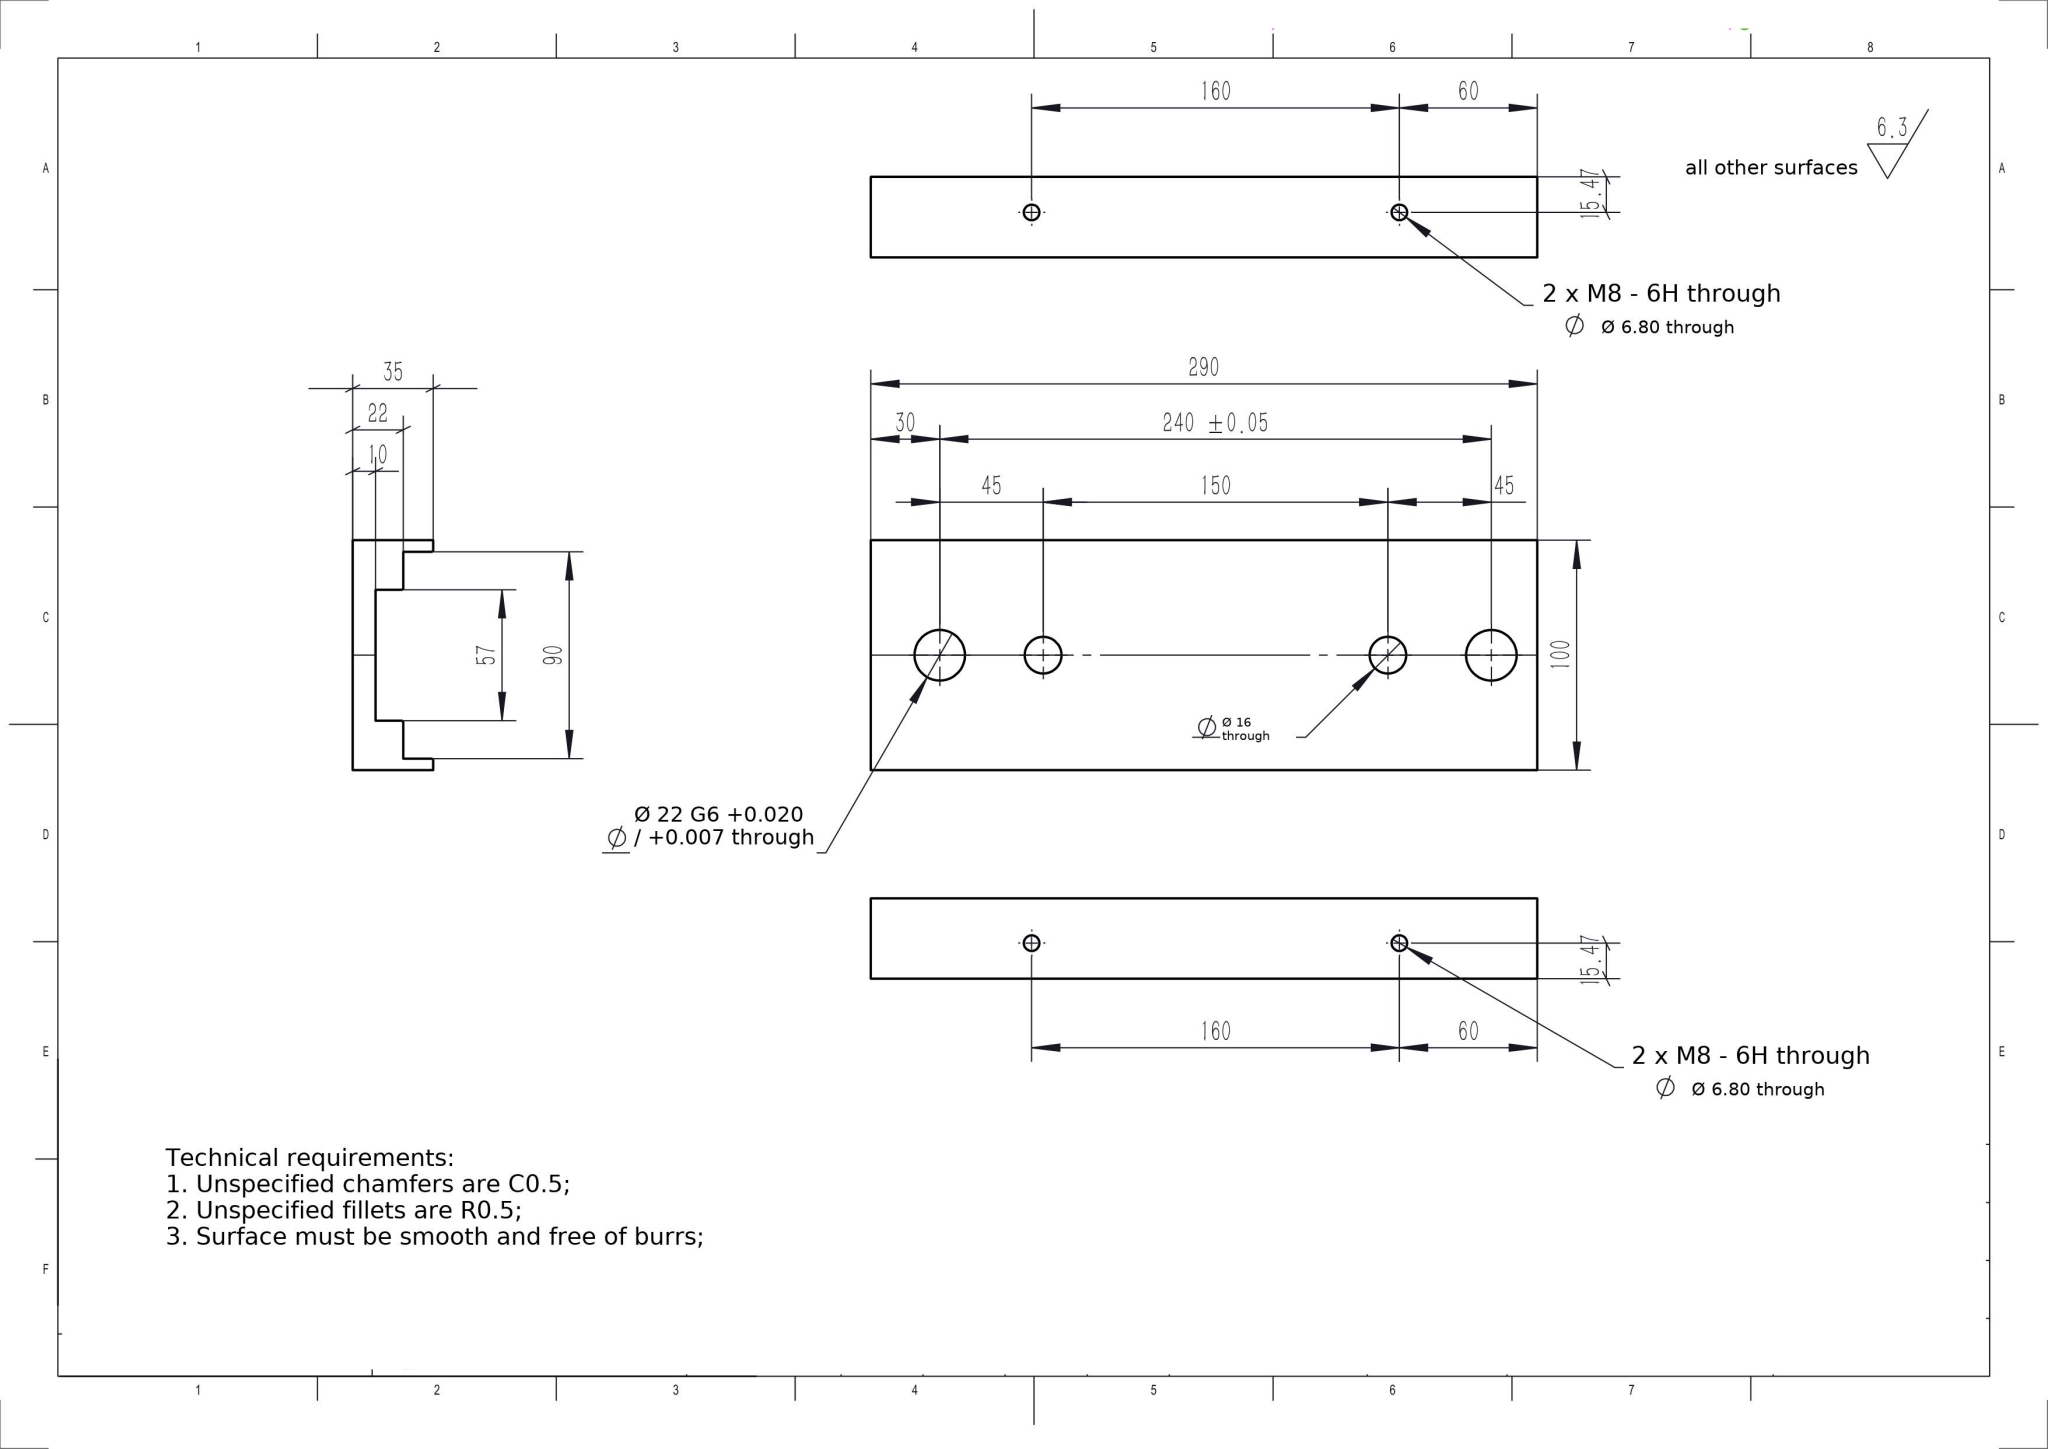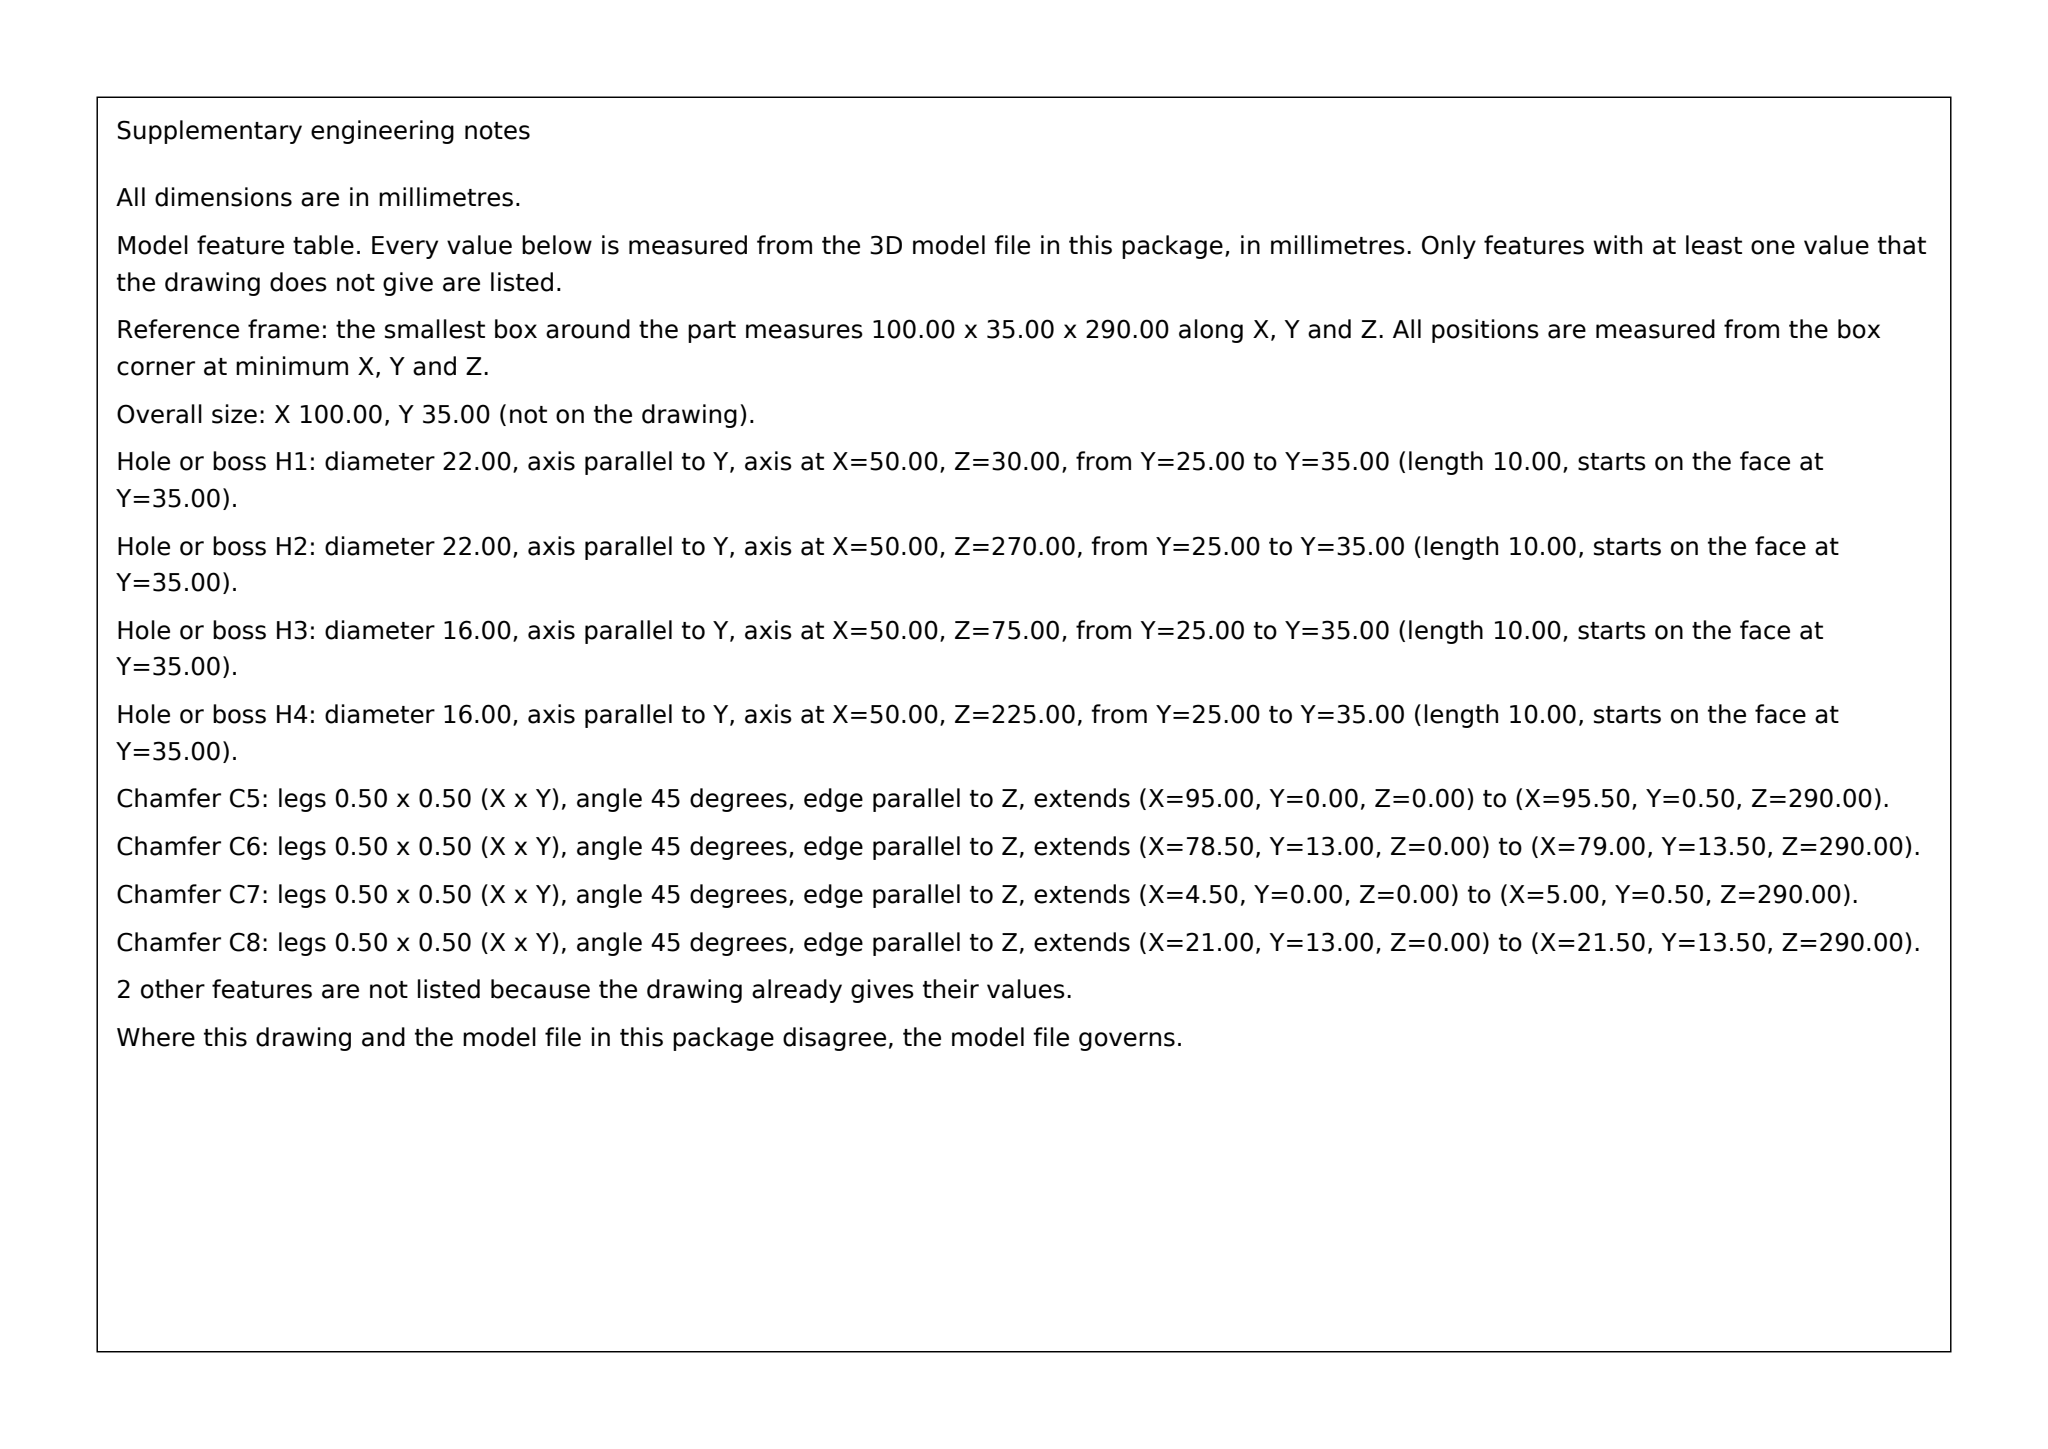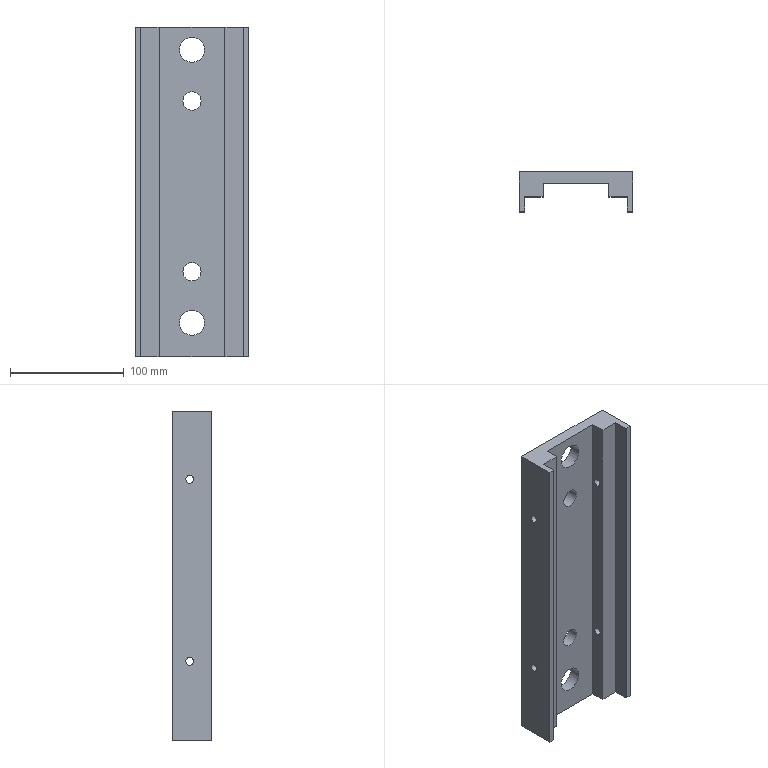Part | SolidWorks | mm | 1 solid | 34 faces | box 100 x 35 x 290 mm | volume 462448 mm3 | plane 18 | cylinder 16 | commonest cylinder face diameters 6.8 x8 22 x4 16 x4
build123d program:
from build123d import *

# Parameters (mm, degrees)
BOSS_EXTRUDE2_DEPTH = 300
SKETCH2_R           = 11
SKETCH2_R_2         = 8
CUT_EXTRUDE1_DEPTH  = 10
M8_TAPPED_HOLE1_D   = 6.8
CHAMFER1_SIZE       = 0.5
SKETCH6_W           = 100
SKETCH6_H           = 10
CUT_EXTRUDE2_DEPTH  = 319.159


with BuildPart() as part:
    # Sketch1 → Boss-Extrude2 (new body)
    with BuildSketch(Plane.XY):
        Polygon((0, 0), (0, 35), (100, 35), (100, 0), (95, 0), (95, 13), (78.5, 13), (78.5, 25), (21.5, 25), (21.5, 13), (5, 13), (5, 0), align=None)
    extrude(amount=BOSS_EXTRUDE2_DEPTH)

    # Sketch2 → Cut-Extrude1 (cut)
    with BuildSketch(Plane(origin=(0, 35, 0), x_dir=(1, 0, 0), z_dir=(0, 1, 0))):
        with Locations(Location((50, -30, 0), (0, 0, 180))):
            Circle(SKETCH2_R)
        with Locations((50, -270)):
            Circle(SKETCH2_R)
        with Locations(Location((50, -75, 0), (0, 0, 180))):
            Circle(SKETCH2_R_2)
        with Locations((50, -225)):
            Circle(SKETCH2_R_2)
    extrude(amount=-CUT_EXTRUDE1_DEPTH, mode=Mode.SUBTRACT)

    # M8 Tapped Hole1 (through all)
    with Locations(Plane(origin=(100, 0, 0), x_dir=(0, 0, -1), z_dir=(1, 0, 0))):
        with Locations((-230, 19.528), (-70, 19.528)):
            Hole(M8_TAPPED_HOLE1_D / 2)

    # Chamfer1
    chamfer1_edges = [part.edges().sort_by_distance(p)[0] for p in [
        (95, 0, 150),
        (78.5, 13, 150),
        (21.5, 13, 150),
        (5, 0, 150),
    ]]
    chamfer(chamfer1_edges, length=CHAMFER1_SIZE)

    # Sketch6 → Cut-Extrude2 (cut, through all)
    with BuildSketch(Plane(origin=(0, 35, 0), x_dir=(1, 0, 0), z_dir=(0, 1, 0))):
        with Locations((50, -295)):
            Rectangle(SKETCH6_W, SKETCH6_H)
    extrude(amount=-CUT_EXTRUDE2_DEPTH, mode=Mode.SUBTRACT)


solid = part.part